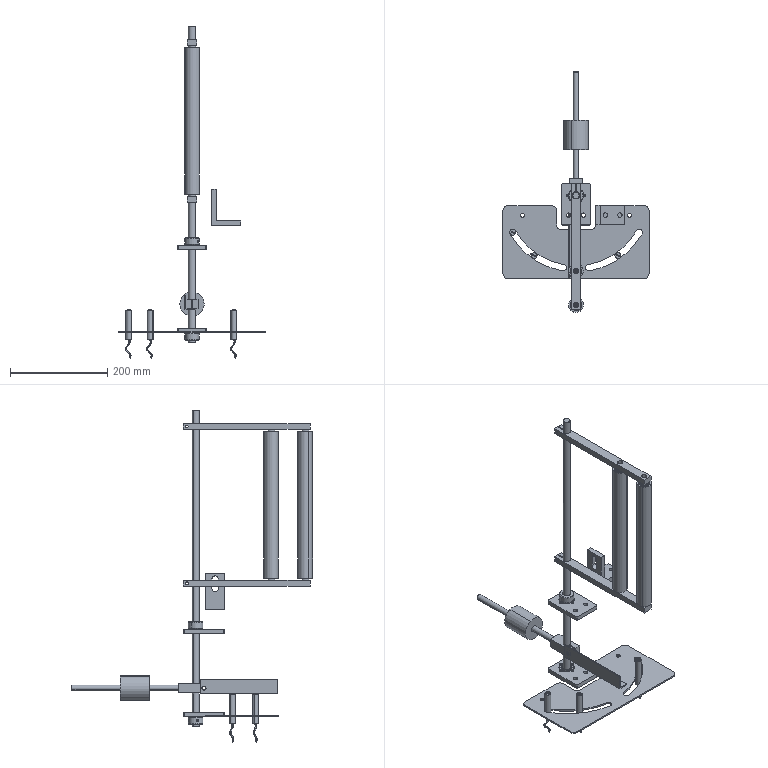Assembly | SolidWorks | mm | 26 component files | 26 solids | 1580 faces | box 300 x 495 x 681.73 mm | volume 1021619 mm3 | sphere 592 | cylinder 328 | plane 322 | torus 288 | cone 44 | spline 6 | commonest cylinder face diameters 15 x34 21.6 x32 5 x20 3.3 x16 24 x16 20 x16 28.8 x16 18.386 x16
Bill of materials:
04_12PhotoelectricSwitch | 3 |  | Slender solid cylindrical body with two small cylindrical studs on one end face and a thin, wavy, curved wire-like strand coming out of the opposite end.
04DeepGrooveBallBearing6002-2Z | 2 |  | Ring-shaped part with concentric inner and outer rings separated by an annular gap. Round rolling elements are visible in the gap, which is consistent with a ball-bearing-like layout.
04DeepGrooveBallBearing61802-2Z | 4 |  | Thin-section ring part with concentric inner and outer rings and many small round elements in the gap between them, a ball-bearing-like layout with a large bore compared with its outer diameter.
KSD171005A-01-01-18 | 1 |  | Long, thin, solid, plain cylindrical rod or pin with flat ends.
KSD171005A-01-01-19 | 2 |  | Flat rectangular plate with chamfered corners, a large circular through hole, four small holes evenly spaced around it, and two medium through holes near the opposite end.
KSD171005A-01-01-20 | 1 |  | Rectangular block with a through bore and a narrow slot running from the bore to one end face, splitting that end, plus a cross hole through the split portion at right angles to the slot. The overall form looks like a split clamp.
KSD171005A-01-01-21 | 1 |  | Solid cylindrical rod or pin with flat ends and slightly broken edges. It is shorter and thicker than unnamed part relative to its length.
KSD171005A-01-01-22 | 1 |  | Thick-walled cylindrical sleeve or spacer with a small central axial through bore.
KSD171005A-01-01-23 | 2 |  | Long rectangular bar with a slotted through bore near one end that splits that end, a small cross hole through the split end, and two smaller through holes spaced along its length.
KSD171005A-01-01-24 | 2 | Chrome Plated Rod | Long, thin cylindrical rod with a small central hole or recess at the end and chamfered end edges.
KSD171005A-01-01-25 | 2 | Aluminum | Straight thin-walled cylindrical tube with an open bore.
KSD171005A-01-01-28 | 2 |  | Short, thick ring or collar with chamfered outer edges, a central through bore, a raised annular step around the bore on one face, and radial holes through the wall.
KSD171005A-01-01-31 | 1 |  | Long, thin, straight L-section (angle) part with two flanges of roughly equal width at 90 degrees, and one small round through-hole near one end of a single flange.
KSD171005A-01-01-32 | 1 |  | Thin flat plate, roughly rectangular, with rounded outer corners, a rectangular notch with rounded corners centered on one long edge, two small round holes near the notched-edge corners, and two arc-shaped slots arranged symmetrically along a common curve.
KSD171005A-01-01-44 | 1 |  | Thick, compact L-bracket (angle block). The base leg has two round through-holes in a row, and the upright leg has one vertically elongated slot with rounded ends.
Mates:
1. concentric | KSD171005A-01-01-18-1 face at (-7.111, 15.73, 978) dir (0, 0, -1) r 7.5 | KSD171005A-01-01-19-1 face at (-7.111, 15.73, 348) dir (0, 0, 1) r 16
2. concentric | KSD171005A-01-01-18-1 face at (-7.111, 15.73, 978) dir (0, 0, -1) r 7.5 | KSD171005A-01-01-19-2 face at (-7.111, 15.73, 528) dir (0, 0, -1) r 16
3. coincident | KSD171005A-01-01-19-1 face at (-37.111, -44.27, 357) dir (0, -1, 0) | KSD171005A-01-01-19-2 face at (22.889, -44.27, 519) dir (0, -1, 0)
4. coincident | KSD171005A-01-01-19-1 face at (-37.111, 40.73, 357) dir (-1, 0, 0) | KSD171005A-01-01-19-2 face at (-37.111, 40.73, 519) dir (-1, 0, 0)
5. concentric | KSD171005A-01-01-18-1 face at (-7.111, 15.73, 978) dir (0, 0, -1) r 7.5 | KSD171005A-01-01-20-1 face at (-7.111, 15.73, 397) dir (0, 0, 1) r 7.5
6. concentric | KSD171005A-01-01-20-1 face at (-7.111, 50.73, 407) dir (0, 1, 0) r 6 | KSD171005A-01-01-21-1 face at (-7.111, 30.73, 407) dir (0, 1, 0) r 6
7. distance | KSD171005A-01-01-20-1 face at (-19.611, 50.73, 417) dir (0, 1, 0) | KSD171005A-01-01-21-1 face at (-7.111, 270.73, 407) dir (0, 1, 0)
8. concentric | KSD171005A-01-01-21-1 face at (-7.111, 30.73, 407) dir (0, 1, 0) r 6 | KSD171005A-01-01-22-1 face at (-7.111, 110.73, 407) dir (0, 1, 0) r 25
9. distance | KSD171005A-01-01-19-1 face at (-7.111, -1.77, 357) dir (0, 0, 1) | KSD171005A-01-01-20-1 face at (-7.111, 15.73, 397) dir (0, 0, -1)
10. concentric | KSD171005A-01-01-18-1 face at (-7.111, 15.73, 978) dir (0, 0, -1) r 7.5 | KSD171005A-01-01-23-1 face at (-7.111, 15.73, 616) dir (0, 0, 1) r 7.5
11. concentric | KSD171005A-01-01-18-1 face at (-7.111, 15.73, 978) dir (0, 0, -1) r 7.5 | KSD171005A-01-01-23-2 face at (-7.111, 15.73, 950) dir (0, 0, -1) r 7.5
12. coincident | KSD171005A-01-01-23-1 face at (-17.111, -219.27, 628) dir (-1, 0, 0) | KSD171005A-01-01-23-2 face at (-17.111, -219.27, 938) dir (-1, 0, 0)
13. concentric | KSD171005A-01-01-23-1 face at (-7.111, -209.27, 616) dir (0, 0, -1) r 3.3 | KSD171005A-01-01-24-1 face at (-7.111, -209.27, 628) dir (0, 0, -1) r 7.5
14. coincident | KSD171005A-01-01-23-1 face at (-7.111, -89.27, 628) dir (0, 0, 1) | KSD171005A-01-01-24-1 face at (-7.111, -209.27, 628) dir (0, 0, -1)
15. coincident | KSD171005A-01-01-23-2 face at (-7.111, -89.27, 938) dir (0, 0, -1) | KSD171005A-01-01-24-1 face at (-11.795, -203.413, 938) dir (0, 0, 1)
16. concentric | KSD171005A-01-01-23-1 face at (-7.111, -139.27, 616) dir (0, 0, -1) r 3.3 | KSD171005A-01-01-24-2 face at (-7.111, -139.27, 628) dir (0, 0, -1) r 7.5
17. coincident | KSD171005A-01-01-23-1 face at (-7.111, -89.27, 628) dir (0, 0, 1) | KSD171005A-01-01-24-2 face at (-7.111, -139.27, 628) dir (0, 0, -1)
18. concentric | KSD171005A-01-01-24-1 face at (-7.111, -209.27, 628) dir (0, 0, -1) r 7.5 | KSD171005A-01-01-25-1 face at (-7.111, -209.27, 589.86) dir (0, 0, -1) r 15
19. coincident | KSD171005A-01-01-24-1 face at (-11.483, -203.803, 633) dir (0, 0, -1) | KSD171005A-01-01-25-1 face at (-13.041, -198.837, 633) dir (0, 0, -1)
20. concentric | KSD171005A-01-01-24-2 face at (-7.111, -139.27, 628) dir (0, 0, -1) r 7.5 | KSD171005A-01-01-25-2 face at (-7.111, -139.27, 589.86) dir (0, 0, -1) r 15
21. coincident | KSD171005A-01-01-24-2 face at (-7.186, -132.271, 633) dir (0, 0, -1) | KSD171005A-01-01-25-2 face at (-18.917, -141.423, 633) dir (0, 0, -1)
22. distance | KSD171005A-01-01-18-1 face at (-7.111, 15.73, 978) dir (0, 0, 1) | KSD171005A-01-01-23-2 face at (-7.111, -89.27, 950) dir (0, 0, 1)
23. distance | KSD171005A-01-01-19-2 face at (-7.111, -1.77, 528) dir (0, 0, 1) | KSD171005A-01-01-19-1 face at (-7.111, -1.77, 348) dir (0, 0, -1)
24. distance | KSD171005A-01-01-21-1 face at (-7.111, 270.73, 407) dir (0, 1, 0) | KSD171005A-01-01-22-1 face at (-7.111, 170.73, 407) dir (0, 1, 0)
25. distance | KSD171005A-01-01-18-1 face at (-7.111, 15.73, 328) dir (0, 0, -1) | KSD171005A-01-01-19-1 face at (-7.111, -1.77, 348) dir (0, 0, -1)
26. concentric | KSD171005A-01-01-18-1 face at (-7.111, 15.73, 978) dir (0, 0, -1) r 7.5 | KSD171005A-01-01-28-1 face at (-7.111, 15.73, 340.5) dir (0, 0, 1) r 7.5
27. coincident | KSD171005A-01-01-19-1 face at (-7.111, -1.77, 348) dir (0, 0, -1) | KSD171005A-01-01-28-1 face at (-8.928, 23.006, 348) dir (0, 0, 1)
28. concentric | KSD171005A-01-01-19-1 face at (-7.111, 15.73, 348) dir (0, 0, 1) r 16 | 04DeepGrooveBallBearing6002-2Z-1 face at (-7.111, 15.73, 352.5) dir (0, 0, -1) r 16
29. coincident | KSD171005A-01-01-19-1 face at (-7.111, -1.77, 348) dir (0, 0, -1) | 04DeepGrooveBallBearing6002-2Z-1 face at (-6.15, 31.4, 348) dir (0, 0, -1)
30. concentric | KSD171005A-01-01-19-2 face at (-7.111, 15.73, 528) dir (0, 0, -1) r 16 | 04DeepGrooveBallBearing6002-2Z-2 face at (-7.111, 15.73, 523.5) dir (0, 0, -1) r 16
31. coincident | KSD171005A-01-01-19-2 face at (-7.111, -1.77, 528) dir (0, 0, 1) | 04DeepGrooveBallBearing6002-2Z-2 face at (-6.15, 31.4, 528) dir (0, 0, 1)
32. concentric | KSD171005A-01-01-18-1 face at (-7.111, 15.73, 978) dir (0, 0, -1) r 7.5 | KSD171005A-01-01-28-2 face at (-7.111, 15.73, 535.5) dir (0, 0, -1) r 15
33. coincident | KSD171005A-01-01-19-2 face at (-7.111, -1.77, 528) dir (0, 0, 1) | KSD171005A-01-01-28-2 face at (-2.778, 21.851, 528) dir (0, 0, -1)
34. concentric | KSD171005A-01-01-25-2 face at (-7.111, -139.27, 589.86) dir (0, 0, -1) r 12 | 04DeepGrooveBallBearing61802-2Z-1 face at (-7.111, -139.27, 635.5) dir (0, 0, -1) r 12
35. coincident | KSD171005A-01-01-25-2 face at (-16.949, -141.064, 638) dir (0, 0, -1) | 04DeepGrooveBallBearing61802-2Z-1 face at (-15.083, -130.706, 638) dir (0, 0, 1)
36. coincident | KSD171005A-01-01-25-2 face at (-18.917, -141.423, 928) dir (0, 0, 1) | 04DeepGrooveBallBearing61802-2Z-2 face at (-15.083, -130.706, 928) dir (0, 0, -1)
37. concentric | KSD171005A-01-01-25-2 face at (-7.111, -139.27, 589.86) dir (0, 0, -1) r 12 | 04DeepGrooveBallBearing61802-2Z-2 face at (-7.111, -139.27, 930.5) dir (0, 0, -1) r 12
38. coincident | KSD171005A-01-01-25-1 face at (-13.041, -198.837, 928) dir (0, 0, 1) | 04DeepGrooveBallBearing61802-2Z-3 face at (-15.083, -200.706, 928) dir (0, 0, -1)
39. concentric | KSD171005A-01-01-25-1 face at (-7.111, -209.27, 589.86) dir (0, 0, -1) r 12 | 04DeepGrooveBallBearing61802-2Z-3 face at (-7.111, -209.27, 930.5) dir (0, 0, -1) r 12
40. coincident | KSD171005A-01-01-25-1 face at (-12.052, -200.576, 638) dir (0, 0, -1) | 04DeepGrooveBallBearing61802-2Z-4 face at (-15.083, -200.706, 638) dir (0, 0, 1)
41. concentric | KSD171005A-01-01-25-1 face at (-7.111, -209.27, 589.86) dir (0, 0, -1) r 12 | 04DeepGrooveBallBearing61802-2Z-4 face at (-7.111, -209.27, 635.5) dir (0, 0, -1) r 12
42. parallel | KSD171005A-01-01-19-2 face at (22.889, 40.73, 519) dir (1, 0, 0) | KSD171005A-01-01-23-1 face at (2.889, -219.27, 628) dir (1, 0, 0)
43. coincident | KSD171005A-01-01-20-1 face at (-19.611, -19.27, 417) dir (-1, 0, 0) | KSD171005A-01-01-31-1 face at (-19.611, 6.73, 425) dir (1, 0, 0)
44. distance | KSD171005A-01-01-32-1 face at (-157.111, -4.27, 351) dir (0, 1, 0) | KSD171005A-01-01-19-1 face at (-37.111, -44.27, 357) dir (0, -1, 0)
45. width | KSD171005A-01-01-19-1 face at (-37.111, 40.73, 357) dir (-1, 0, 0) | KSD171005A-01-01-19-1 face at (22.889, 40.73, 357) dir (1, 0, 0) | KSD171005A-01-01-32-1 face at (-157.111, -154.27, 351) dir (-1, 0, 0) | KSD171005A-01-01-32-1 face at (142.889, -154.27, 351) dir (1, 0, 0)
46. coincident | KSD171005A-01-01-19-1 face at (-7.111, -1.77, 348) dir (0, 0, -1) | KSD171005A-01-01-32-1 face at (-7.111, -79.27, 348) dir (0, 0, -1)
47. concentric | KSD171005A-01-01-20-1 face at (-19.611, -1.27, 407) dir (-1, 0, 0) r 4.25 | KSD171005A-01-01-31-1 face at (-21.611, -1.27, 407) dir (-1, 0, 0) r 4.25
48. parallel | KSD171005A-01-01-20-1 face at (-7.111, 15.73, 417) dir (0, 0, 1) | KSD171005A-01-01-31-1 face at (-19.611, 6.73, 425) dir (0, 0, 1)
49. concentric | KSD171005A-01-01-32-1 face at (-137.015, -59.27, 341) dir (0, 0, 1) r 6.5 | 04_12PhotoelectricSwitch-1 face at (-137.015, -59.27, 394) dir (0, 0, -1) r 6
50. concentric | KSD171005A-01-01-32-1 axis at (-93.148, -107.143, 348) dir (0, 0, 1) | 04_12PhotoelectricSwitch-2 face at (-93.148, -107.143, 394) dir (0, 0, -1) r 6
51. concentric | KSD171005A-01-01-32-1 axis at (78.925, -107.143, 348) dir (0, 0, 1) | 04_12PhotoelectricSwitch-3 face at (78.925, -107.143, 394) dir (0, 0, -1) r 6
52. coincident | 04_12PhotoelectricSwitch-1 face at (-137.015, -59.27, 394) dir (0, 0, 1) | 04_12PhotoelectricSwitch-2 face at (-93.148, -107.143, 394) dir (0, 0, 1)
53. coincident | 04_12PhotoelectricSwitch-2 face at (-93.148, -107.143, 394) dir (0, 0, 1) | 04_12PhotoelectricSwitch-3 face at (78.925, -107.143, 394) dir (0, 0, 1)
54. coincident | KSD171005A-01-01-31-1 face at (-21.611, 6.73, 395) dir (0, 0, -1) | 04_12PhotoelectricSwitch-2 face at (-95.095, -106.015, 395) dir (0, 0, 1)
55. parallel | KSD171005A-01-01-19-1 face at (-37.111, 40.73, 357) dir (-1, 0, 0) | KSD171005A-01-01-20-1 face at (-19.611, -19.27, 417) dir (-1, 0, 0)
56. coincident | KSD171005A-01-01-19-2 face at (22.889, -44.27, 519) dir (0, -1, 0) | KSD171005A-01-01-44-1 face at (32.889, -44.27, 568) dir (0, -1, 0)
57. distance | KSD171005A-01-01-19-2 face at (-7.111, -1.77, 528) dir (0, 0, 1) | KSD171005A-01-01-44-1 face at (32.889, -44.27, 568) dir (0, 0, -1)
58. distance | KSD171005A-01-01-23-1 face at (2.889, -219.27, 628) dir (1, 0, 0) | KSD171005A-01-01-44-1 face at (32.889, -44.27, 568) dir (-1, 0, 0)